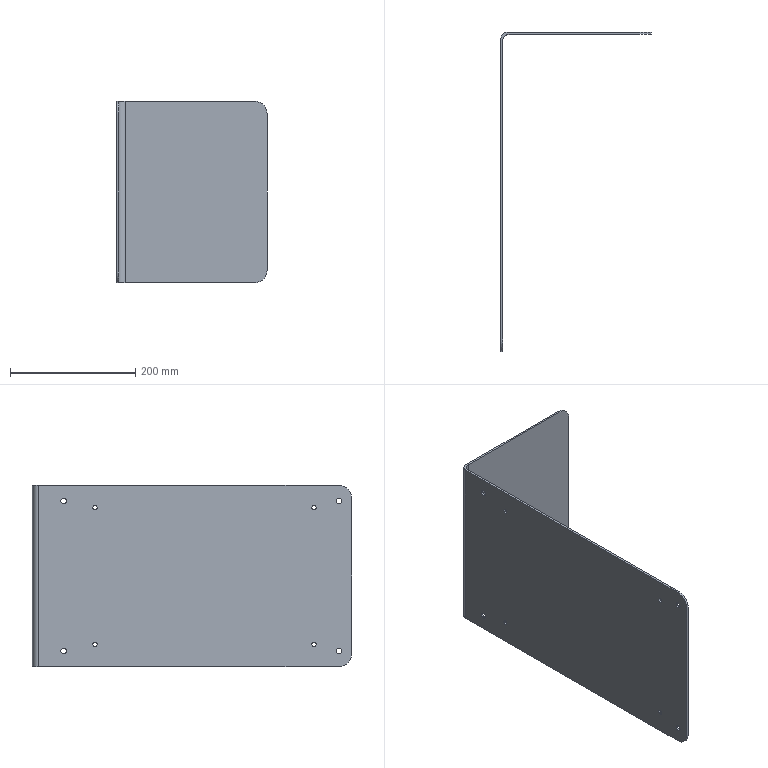Component | SolidWorks | 200-250InverterBracket()-1 | 1 solid | 30 faces | box 240 x 510 x 290 mm | volume 647635 mm3 | cylinder 22 | plane 8 | commonest cylinder face diameters 7 x8 9 x8 40 x4 20 x2 | material Plain Carbon Steel
STEP:
#1=COLOUR_RGB('',0.7922,0.8196,0.9333);
#2=FILL_AREA_STYLE_COLOUR('',#1);
#3=FILL_AREA_STYLE('',(#2));
#4=SURFACE_STYLE_FILL_AREA(#3);
#5=SURFACE_SIDE_STYLE('',(#4));
#6=SURFACE_STYLE_USAGE(.BOTH.,#5);
#7=PRESENTATION_STYLE_ASSIGNMENT((#6));
#8=CARTESIAN_POINT('',(26.575,78.996,-60.669));
#9=VERTEX_POINT('',#8);
#10=CARTESIAN_POINT('',(26.575,79.272,-60.669));
#11=VERTEX_POINT('',#10);
#12=CARTESIAN_POINT('',(26.575,79.134,-60.669));
#13=DIRECTION('',(-1.,0.,-0.));
#14=DIRECTION('',(0.,-1.,0.));
#15=AXIS2_PLACEMENT_3D('',#12,#13,#14);
#16=CIRCLE('',#15,0.1378);
#17=EDGE_CURVE('',#9,#11,#16,.T.);
#18=ORIENTED_EDGE('',*,*,#17,.T.);
#19=CARTESIAN_POINT('',(26.693,79.272,-60.669));
#20=VERTEX_POINT('',#19);
#21=CARTESIAN_POINT('',(26.693,79.272,-60.669));
#22=DIRECTION('',(1.,-0.,0.));
#23=VECTOR('',#22,39.37);
#24=LINE('',#21,#23);
#25=EDGE_CURVE('',#11,#20,#24,.T.);
#26=ORIENTED_EDGE('',*,*,#25,.T.);
#27=CARTESIAN_POINT('',(26.693,78.996,-60.669));
#28=VERTEX_POINT('',#27);
#29=CARTESIAN_POINT('',(26.693,79.134,-60.669));
#30=DIRECTION('',(-1.,0.,-0.));
#31=DIRECTION('',(0.,-1.,0.));
#32=AXIS2_PLACEMENT_3D('',#29,#30,#31);
#33=CIRCLE('',#32,0.1378);
#34=EDGE_CURVE('',#28,#20,#33,.T.);
#35=ORIENTED_EDGE('',*,*,#34,.F.);
#36=CARTESIAN_POINT('',(26.693,78.996,-60.669));
#37=DIRECTION('',(1.,-0.,0.));
#38=VECTOR('',#37,39.37);
#39=LINE('',#36,#38);
#40=EDGE_CURVE('',#9,#28,#39,.T.);
#41=ORIENTED_EDGE('',*,*,#40,.F.);
#42=EDGE_LOOP('',(#18,#26,#35,#41));
#43=FACE_OUTER_BOUND('',#42,.T.);
#44=CARTESIAN_POINT('',(26.693,79.134,-60.669));
#45=DIRECTION('',(1.,-0.,0.));
#46=DIRECTION('',(0.,-1.,0.));
#47=AXIS2_PLACEMENT_3D('',#44,#45,#46);
#48=CYLINDRICAL_SURFACE('',#47,0.1378);
#49=ADVANCED_FACE('',(#43),#48,.F.);
#50=CARTESIAN_POINT('',(26.575,78.996,-69.252));
#51=VERTEX_POINT('',#50);
#52=CARTESIAN_POINT('',(26.575,79.272,-69.252));
#53=VERTEX_POINT('',#52);
#54=CARTESIAN_POINT('',(26.575,79.134,-69.252));
#55=DIRECTION('',(-1.,0.,-0.));
#56=DIRECTION('',(0.,-1.,0.));
#57=AXIS2_PLACEMENT_3D('',#54,#55,#56);
#58=CIRCLE('',#57,0.1378);
#59=EDGE_CURVE('',#51,#53,#58,.T.);
#60=ORIENTED_EDGE('',*,*,#59,.T.);
#61=CARTESIAN_POINT('',(26.693,79.272,-69.252));
#62=VERTEX_POINT('',#61);
#63=CARTESIAN_POINT('',(26.693,79.272,-69.252));
#64=DIRECTION('',(1.,-0.,0.));
#65=VECTOR('',#64,39.37);
#66=LINE('',#63,#65);
#67=EDGE_CURVE('',#53,#62,#66,.T.);
#68=ORIENTED_EDGE('',*,*,#67,.T.);
#69=CARTESIAN_POINT('',(26.693,78.996,-69.252));
#70=VERTEX_POINT('',#69);
#71=CARTESIAN_POINT('',(26.693,79.134,-69.252));
#72=DIRECTION('',(-1.,0.,-0.));
#73=DIRECTION('',(0.,-1.,0.));
#74=AXIS2_PLACEMENT_3D('',#71,#72,#73);
#75=CIRCLE('',#74,0.1378);
#76=EDGE_CURVE('',#70,#62,#75,.T.);
#77=ORIENTED_EDGE('',*,*,#76,.F.);
#78=CARTESIAN_POINT('',(26.693,78.996,-69.252));
#79=DIRECTION('',(1.,-0.,0.));
#80=VECTOR('',#79,39.37);
#81=LINE('',#78,#80);
#82=EDGE_CURVE('',#51,#70,#81,.T.);
#83=ORIENTED_EDGE('',*,*,#82,.F.);
#84=EDGE_LOOP('',(#60,#68,#77,#83));
#85=FACE_OUTER_BOUND('',#84,.T.);
#86=CARTESIAN_POINT('',(26.693,79.134,-69.252));
#87=DIRECTION('',(1.,-0.,0.));
#88=DIRECTION('',(0.,-1.,0.));
#89=AXIS2_PLACEMENT_3D('',#86,#87,#88);
#90=CYLINDRICAL_SURFACE('',#89,0.1378);
#91=ADVANCED_FACE('',(#85),#90,.F.);
#92=CARTESIAN_POINT('',(26.575,92.776,-69.252));
#93=VERTEX_POINT('',#92);
#94=CARTESIAN_POINT('',(26.575,93.051,-69.252));
#95=VERTEX_POINT('',#94);
#96=CARTESIAN_POINT('',(26.575,92.913,-69.252));
#97=DIRECTION('',(-1.,0.,-0.));
#98=DIRECTION('',(0.,-1.,0.));
#99=AXIS2_PLACEMENT_3D('',#96,#97,#98);
#100=CIRCLE('',#99,0.1378);
#101=EDGE_CURVE('',#93,#95,#100,.T.);
#102=ORIENTED_EDGE('',*,*,#101,.T.);
#103=CARTESIAN_POINT('',(26.693,93.051,-69.252));
#104=VERTEX_POINT('',#103);
#105=CARTESIAN_POINT('',(26.693,93.051,-69.252));
#106=DIRECTION('',(1.,-0.,0.));
#107=VECTOR('',#106,39.37);
#108=LINE('',#105,#107);
#109=EDGE_CURVE('',#95,#104,#108,.T.);
#110=ORIENTED_EDGE('',*,*,#109,.T.);
#111=CARTESIAN_POINT('',(26.693,92.776,-69.252));
#112=VERTEX_POINT('',#111);
#113=CARTESIAN_POINT('',(26.693,92.913,-69.252));
#114=DIRECTION('',(-1.,0.,-0.));
#115=DIRECTION('',(0.,-1.,0.));
#116=AXIS2_PLACEMENT_3D('',#113,#114,#115);
#117=CIRCLE('',#116,0.1378);
#118=EDGE_CURVE('',#112,#104,#117,.T.);
#119=ORIENTED_EDGE('',*,*,#118,.F.);
#120=CARTESIAN_POINT('',(26.693,92.776,-69.252));
#121=DIRECTION('',(1.,-0.,0.));
#122=VECTOR('',#121,39.37);
#123=LINE('',#120,#122);
#124=EDGE_CURVE('',#93,#112,#123,.T.);
#125=ORIENTED_EDGE('',*,*,#124,.F.);
#126=EDGE_LOOP('',(#102,#110,#119,#125));
#127=FACE_OUTER_BOUND('',#126,.T.);
#128=CARTESIAN_POINT('',(26.693,92.913,-69.252));
#129=DIRECTION('',(1.,-0.,0.));
#130=DIRECTION('',(0.,-1.,0.));
#131=AXIS2_PLACEMENT_3D('',#128,#129,#130);
#132=CYLINDRICAL_SURFACE('',#131,0.1378);
#133=ADVANCED_FACE('',(#127),#132,.F.);
#134=CARTESIAN_POINT('',(26.575,92.776,-60.669));
#135=VERTEX_POINT('',#134);
#136=CARTESIAN_POINT('',(26.575,93.051,-60.669));
#137=VERTEX_POINT('',#136);
#138=CARTESIAN_POINT('',(26.575,92.913,-60.669));
#139=DIRECTION('',(-1.,0.,-0.));
#140=DIRECTION('',(0.,-1.,0.));
#141=AXIS2_PLACEMENT_3D('',#138,#139,#140);
#142=CIRCLE('',#141,0.1378);
#143=EDGE_CURVE('',#135,#137,#142,.T.);
#144=ORIENTED_EDGE('',*,*,#143,.T.);
#145=CARTESIAN_POINT('',(26.693,93.051,-60.669));
#146=VERTEX_POINT('',#145);
#147=CARTESIAN_POINT('',(26.693,93.051,-60.669));
#148=DIRECTION('',(1.,-0.,0.));
#149=VECTOR('',#148,39.37);
#150=LINE('',#147,#149);
#151=EDGE_CURVE('',#137,#146,#150,.T.);
#152=ORIENTED_EDGE('',*,*,#151,.T.);
#153=CARTESIAN_POINT('',(26.693,92.776,-60.669));
#154=VERTEX_POINT('',#153);
#155=CARTESIAN_POINT('',(26.693,92.913,-60.669));
#156=DIRECTION('',(-1.,0.,-0.));
#157=DIRECTION('',(0.,-1.,0.));
#158=AXIS2_PLACEMENT_3D('',#155,#156,#157);
#159=CIRCLE('',#158,0.1378);
#160=EDGE_CURVE('',#154,#146,#159,.T.);
#161=ORIENTED_EDGE('',*,*,#160,.F.);
#162=CARTESIAN_POINT('',(26.693,92.776,-60.669));
#163=DIRECTION('',(1.,-0.,0.));
#164=VECTOR('',#163,39.37);
#165=LINE('',#162,#164);
#166=EDGE_CURVE('',#135,#154,#165,.T.);
#167=ORIENTED_EDGE('',*,*,#166,.F.);
#168=EDGE_LOOP('',(#144,#152,#161,#167));
#169=FACE_OUTER_BOUND('',#168,.T.);
#170=CARTESIAN_POINT('',(26.693,92.913,-60.669));
#171=DIRECTION('',(1.,-0.,0.));
#172=DIRECTION('',(0.,-1.,0.));
#173=AXIS2_PLACEMENT_3D('',#170,#171,#172);
#174=CYLINDRICAL_SURFACE('',#173,0.1378);
#175=ADVANCED_FACE('',(#169),#174,.F.);
#176=CARTESIAN_POINT('',(26.575,77.382,-69.685));
#177=VERTEX_POINT('',#176);
#178=CARTESIAN_POINT('',(26.575,77.736,-69.685));
#179=VERTEX_POINT('',#178);
#180=CARTESIAN_POINT('',(26.575,77.559,-69.685));
#181=DIRECTION('',(-1.,0.,-0.));
#182=DIRECTION('',(0.,-1.,0.));
#183=AXIS2_PLACEMENT_3D('',#180,#181,#182);
#184=CIRCLE('',#183,0.1772);
#185=EDGE_CURVE('',#177,#179,#184,.T.);
#186=ORIENTED_EDGE('',*,*,#185,.T.);
#187=CARTESIAN_POINT('',(26.693,77.736,-69.685));
#188=VERTEX_POINT('',#187);
#189=CARTESIAN_POINT('',(26.693,77.736,-69.685));
#190=DIRECTION('',(1.,-0.,0.));
#191=VECTOR('',#190,39.37);
#192=LINE('',#189,#191);
#193=EDGE_CURVE('',#179,#188,#192,.T.);
#194=ORIENTED_EDGE('',*,*,#193,.T.);
#195=CARTESIAN_POINT('',(26.693,77.382,-69.685));
#196=VERTEX_POINT('',#195);
#197=CARTESIAN_POINT('',(26.693,77.559,-69.685));
#198=DIRECTION('',(-1.,0.,-0.));
#199=DIRECTION('',(0.,-1.,0.));
#200=AXIS2_PLACEMENT_3D('',#197,#198,#199);
#201=CIRCLE('',#200,0.1772);
#202=EDGE_CURVE('',#196,#188,#201,.T.);
#203=ORIENTED_EDGE('',*,*,#202,.F.);
#204=CARTESIAN_POINT('',(26.693,77.382,-69.685));
#205=DIRECTION('',(1.,-0.,0.));
#206=VECTOR('',#205,39.37);
#207=LINE('',#204,#206);
#208=EDGE_CURVE('',#177,#196,#207,.T.);
#209=ORIENTED_EDGE('',*,*,#208,.F.);
#210=EDGE_LOOP('',(#186,#194,#203,#209));
#211=FACE_OUTER_BOUND('',#210,.T.);
#212=CARTESIAN_POINT('',(26.693,77.559,-69.685));
#213=DIRECTION('',(1.,-0.,0.));
#214=DIRECTION('',(0.,-1.,0.));
#215=AXIS2_PLACEMENT_3D('',#212,#213,#214);
#216=CYLINDRICAL_SURFACE('',#215,0.1772);
#217=ADVANCED_FACE('',(#211),#216,.F.);
#218=CARTESIAN_POINT('',(26.575,77.382,-60.236));
#219=VERTEX_POINT('',#218);
#220=CARTESIAN_POINT('',(26.575,77.736,-60.236));
#221=VERTEX_POINT('',#220);
#222=CARTESIAN_POINT('',(26.575,77.559,-60.236));
#223=DIRECTION('',(-1.,0.,-0.));
#224=DIRECTION('',(0.,-1.,0.));
#225=AXIS2_PLACEMENT_3D('',#222,#223,#224);
#226=CIRCLE('',#225,0.1772);
#227=EDGE_CURVE('',#219,#221,#226,.T.);
#228=ORIENTED_EDGE('',*,*,#227,.T.);
#229=CARTESIAN_POINT('',(26.693,77.736,-60.236));
#230=VERTEX_POINT('',#229);
#231=CARTESIAN_POINT('',(26.693,77.736,-60.236));
#232=DIRECTION('',(1.,-0.,0.));
#233=VECTOR('',#232,39.37);
#234=LINE('',#231,#233);
#235=EDGE_CURVE('',#221,#230,#234,.T.);
#236=ORIENTED_EDGE('',*,*,#235,.T.);
#237=CARTESIAN_POINT('',(26.693,77.382,-60.236));
#238=VERTEX_POINT('',#237);
#239=CARTESIAN_POINT('',(26.693,77.559,-60.236));
#240=DIRECTION('',(-1.,0.,-0.));
#241=DIRECTION('',(0.,-1.,0.));
#242=AXIS2_PLACEMENT_3D('',#239,#240,#241);
#243=CIRCLE('',#242,0.1772);
#244=EDGE_CURVE('',#238,#230,#243,.T.);
#245=ORIENTED_EDGE('',*,*,#244,.F.);
#246=CARTESIAN_POINT('',(26.693,77.382,-60.236));
#247=DIRECTION('',(1.,-0.,0.));
#248=VECTOR('',#247,39.37);
#249=LINE('',#246,#248);
#250=EDGE_CURVE('',#219,#238,#249,.T.);
#251=ORIENTED_EDGE('',*,*,#250,.F.);
#252=EDGE_LOOP('',(#228,#236,#245,#251));
#253=FACE_OUTER_BOUND('',#252,.T.);
#254=CARTESIAN_POINT('',(26.693,77.559,-60.236));
#255=DIRECTION('',(1.,-0.,0.));
#256=DIRECTION('',(0.,-1.,0.));
#257=AXIS2_PLACEMENT_3D('',#254,#255,#256);
#258=CYLINDRICAL_SURFACE('',#257,0.1772);
#259=ADVANCED_FACE('',(#253),#258,.F.);
#260=CARTESIAN_POINT('',(26.575,94.705,-60.236));
#261=VERTEX_POINT('',#260);
#262=CARTESIAN_POINT('',(26.575,95.059,-60.236));
#263=VERTEX_POINT('',#262);
#264=CARTESIAN_POINT('',(26.575,94.882,-60.236));
#265=DIRECTION('',(-1.,0.,-0.));
#266=DIRECTION('',(0.,-1.,0.));
#267=AXIS2_PLACEMENT_3D('',#264,#265,#266);
#268=CIRCLE('',#267,0.1772);
#269=EDGE_CURVE('',#261,#263,#268,.T.);
#270=ORIENTED_EDGE('',*,*,#269,.T.);
#271=CARTESIAN_POINT('',(26.693,95.059,-60.236));
#272=VERTEX_POINT('',#271);
#273=CARTESIAN_POINT('',(26.693,95.059,-60.236));
#274=DIRECTION('',(1.,-0.,0.));
#275=VECTOR('',#274,39.37);
#276=LINE('',#273,#275);
#277=EDGE_CURVE('',#263,#272,#276,.T.);
#278=ORIENTED_EDGE('',*,*,#277,.T.);
#279=CARTESIAN_POINT('',(26.693,94.705,-60.236));
#280=VERTEX_POINT('',#279);
#281=CARTESIAN_POINT('',(26.693,94.882,-60.236));
#282=DIRECTION('',(-1.,0.,-0.));
#283=DIRECTION('',(0.,-1.,0.));
#284=AXIS2_PLACEMENT_3D('',#281,#282,#283);
#285=CIRCLE('',#284,0.1772);
#286=EDGE_CURVE('',#280,#272,#285,.T.);
#287=ORIENTED_EDGE('',*,*,#286,.F.);
#288=CARTESIAN_POINT('',(26.693,94.705,-60.236));
#289=DIRECTION('',(1.,-0.,0.));
#290=VECTOR('',#289,39.37);
#291=LINE('',#288,#290);
#292=EDGE_CURVE('',#261,#280,#291,.T.);
#293=ORIENTED_EDGE('',*,*,#292,.F.);
#294=EDGE_LOOP('',(#270,#278,#287,#293));
#295=FACE_OUTER_BOUND('',#294,.T.);
#296=CARTESIAN_POINT('',(26.693,94.882,-60.236));
#297=DIRECTION('',(1.,-0.,0.));
#298=DIRECTION('',(0.,-1.,0.));
#299=AXIS2_PLACEMENT_3D('',#296,#297,#298);
#300=CYLINDRICAL_SURFACE('',#299,0.1772);
#301=ADVANCED_FACE('',(#295),#300,.F.);
#302=CARTESIAN_POINT('',(26.575,94.705,-69.685));
#303=VERTEX_POINT('',#302);
#304=CARTESIAN_POINT('',(26.575,95.059,-69.685));
#305=VERTEX_POINT('',#304);
#306=CARTESIAN_POINT('',(26.575,94.882,-69.685));
#307=DIRECTION('',(-1.,0.,-0.));
#308=DIRECTION('',(0.,-1.,0.));
#309=AXIS2_PLACEMENT_3D('',#306,#307,#308);
#310=CIRCLE('',#309,0.1772);
#311=EDGE_CURVE('',#303,#305,#310,.T.);
#312=ORIENTED_EDGE('',*,*,#311,.T.);
#313=CARTESIAN_POINT('',(26.693,95.059,-69.685));
#314=VERTEX_POINT('',#313);
#315=CARTESIAN_POINT('',(26.693,95.059,-69.685));
#316=DIRECTION('',(1.,-0.,0.));
#317=VECTOR('',#316,39.37);
#318=LINE('',#315,#317);
#319=EDGE_CURVE('',#305,#314,#318,.T.);
#320=ORIENTED_EDGE('',*,*,#319,.T.);
#321=CARTESIAN_POINT('',(26.693,94.705,-69.685));
#322=VERTEX_POINT('',#321);
#323=CARTESIAN_POINT('',(26.693,94.882,-69.685));
#324=DIRECTION('',(-1.,0.,-0.));
#325=DIRECTION('',(0.,-1.,0.));
#326=AXIS2_PLACEMENT_3D('',#323,#324,#325);
#327=CIRCLE('',#326,0.1772);
#328=EDGE_CURVE('',#322,#314,#327,.T.);
#329=ORIENTED_EDGE('',*,*,#328,.F.);
#330=CARTESIAN_POINT('',(26.693,94.705,-69.685));
#331=DIRECTION('',(1.,-0.,0.));
#332=VECTOR('',#331,39.37);
#333=LINE('',#330,#332);
#334=EDGE_CURVE('',#303,#322,#333,.T.);
#335=ORIENTED_EDGE('',*,*,#334,.F.);
#336=EDGE_LOOP('',(#312,#320,#329,#335));
#337=FACE_OUTER_BOUND('',#336,.T.);
#338=CARTESIAN_POINT('',(26.693,94.882,-69.685));
#339=DIRECTION('',(1.,-0.,0.));
#340=DIRECTION('',(0.,-1.,0.));
#341=AXIS2_PLACEMENT_3D('',#338,#339,#340);
#342=CYLINDRICAL_SURFACE('',#341,0.1772);
#343=ADVANCED_FACE('',(#337),#342,.F.);
#344=CARTESIAN_POINT('',(26.575,76.772,-69.882));
#345=VERTEX_POINT('',#344);
#346=CARTESIAN_POINT('',(26.575,77.559,-70.669));
#347=VERTEX_POINT('',#346);
#348=CARTESIAN_POINT('',(26.575,77.559,-69.882));
#349=DIRECTION('',(1.,-0.,0.));
#350=DIRECTION('',(0.,-1.,0.));
#351=AXIS2_PLACEMENT_3D('',#348,#349,#350);
#352=CIRCLE('',#351,0.7874);
#353=EDGE_CURVE('',#345,#347,#352,.T.);
#354=ORIENTED_EDGE('',*,*,#353,.F.);
#355=CARTESIAN_POINT('',(26.575,76.772,-60.039));
#356=VERTEX_POINT('',#355);
#357=CARTESIAN_POINT('',(26.575,76.772,-70.669));
#358=DIRECTION('',(0.,0.,-1.));
#359=VECTOR('',#358,39.37);
#360=LINE('',#357,#359);
#361=EDGE_CURVE('',#356,#345,#360,.T.);
#362=ORIENTED_EDGE('',*,*,#361,.F.);
#363=CARTESIAN_POINT('',(26.575,77.559,-59.252));
#364=VERTEX_POINT('',#363);
#365=CARTESIAN_POINT('',(26.575,77.559,-60.039));
#366=DIRECTION('',(1.,-0.,0.));
#367=DIRECTION('',(0.,1.,0.));
#368=AXIS2_PLACEMENT_3D('',#365,#366,#367);
#369=CIRCLE('',#368,0.7874);
#370=EDGE_CURVE('',#364,#356,#369,.T.);
#371=ORIENTED_EDGE('',*,*,#370,.F.);
#372=CARTESIAN_POINT('',(26.575,96.457,-59.252));
#373=VERTEX_POINT('',#372);
#374=CARTESIAN_POINT('',(26.575,76.772,-59.252));
#375=DIRECTION('',(-0.,-1.,-0.));
#376=VECTOR('',#375,39.37);
#377=LINE('',#374,#376);
#378=EDGE_CURVE('',#373,#364,#377,.T.);
#379=ORIENTED_EDGE('',*,*,#378,.F.);
#380=CARTESIAN_POINT('',(26.575,96.457,-70.669));
#381=VERTEX_POINT('',#380);
#382=CARTESIAN_POINT('',(26.575,96.457,-70.669));
#383=DIRECTION('',(-0.,-0.,1.));
#384=VECTOR('',#383,39.37);
#385=LINE('',#382,#384);
#386=EDGE_CURVE('',#381,#373,#385,.T.);
#387=ORIENTED_EDGE('',*,*,#386,.F.);
#388=CARTESIAN_POINT('',(26.575,76.772,-70.669));
#389=DIRECTION('',(0.,1.,0.));
#390=VECTOR('',#389,39.37);
#391=LINE('',#388,#390);
#392=EDGE_CURVE('',#347,#381,#391,.T.);
#393=ORIENTED_EDGE('',*,*,#392,.F.);
#394=EDGE_LOOP('',(#354,#362,#371,#379,#387,#393));
#395=FACE_OUTER_BOUND('',#394,.T.);
#396=ORIENTED_EDGE('',*,*,#17,.F.);
#397=CARTESIAN_POINT('',(26.575,79.134,-60.669));
#398=DIRECTION('',(-1.,0.,-0.));
#399=DIRECTION('',(0.,-1.,0.));
#400=AXIS2_PLACEMENT_3D('',#397,#398,#399);
#401=CIRCLE('',#400,0.1378);
#402=EDGE_CURVE('',#11,#9,#401,.T.);
#403=ORIENTED_EDGE('',*,*,#402,.F.);
#404=EDGE_LOOP('',(#396,#403));
#405=FACE_BOUND('',#404,.T.);
#406=ORIENTED_EDGE('',*,*,#59,.F.);
#407=CARTESIAN_POINT('',(26.575,79.134,-69.252));
#408=DIRECTION('',(-1.,0.,-0.));
#409=DIRECTION('',(0.,-1.,0.));
#410=AXIS2_PLACEMENT_3D('',#407,#408,#409);
#411=CIRCLE('',#410,0.1378);
#412=EDGE_CURVE('',#53,#51,#411,.T.);
#413=ORIENTED_EDGE('',*,*,#412,.F.);
#414=EDGE_LOOP('',(#406,#413));
#415=FACE_BOUND('',#414,.T.);
#416=ORIENTED_EDGE('',*,*,#101,.F.);
#417=CARTESIAN_POINT('',(26.575,92.913,-69.252));
#418=DIRECTION('',(-1.,0.,-0.));
#419=DIRECTION('',(0.,-1.,0.));
#420=AXIS2_PLACEMENT_3D('',#417,#418,#419);
#421=CIRCLE('',#420,0.1378);
#422=EDGE_CURVE('',#95,#93,#421,.T.);
#423=ORIENTED_EDGE('',*,*,#422,.F.);
#424=EDGE_LOOP('',(#416,#423));
#425=FACE_BOUND('',#424,.T.);
#426=ORIENTED_EDGE('',*,*,#143,.F.);
#427=CARTESIAN_POINT('',(26.575,92.913,-60.669));
#428=DIRECTION('',(-1.,0.,-0.));
#429=DIRECTION('',(0.,-1.,0.));
#430=AXIS2_PLACEMENT_3D('',#427,#428,#429);
#431=CIRCLE('',#430,0.1378);
#432=EDGE_CURVE('',#137,#135,#431,.T.);
#433=ORIENTED_EDGE('',*,*,#432,.F.);
#434=EDGE_LOOP('',(#426,#433));
#435=FACE_BOUND('',#434,.T.);
#436=ORIENTED_EDGE('',*,*,#185,.F.);
#437=CARTESIAN_POINT('',(26.575,77.559,-69.685));
#438=DIRECTION('',(-1.,0.,-0.));
#439=DIRECTION('',(0.,-1.,0.));
#440=AXIS2_PLACEMENT_3D('',#437,#438,#439);
#441=CIRCLE('',#440,0.1772);
#442=EDGE_CURVE('',#179,#177,#441,.T.);
#443=ORIENTED_EDGE('',*,*,#442,.F.);
#444=EDGE_LOOP('',(#436,#443));
#445=FACE_BOUND('',#444,.T.);
#446=ORIENTED_EDGE('',*,*,#227,.F.);
#447=CARTESIAN_POINT('',(26.575,77.559,-60.236));
#448=DIRECTION('',(-1.,0.,-0.));
#449=DIRECTION('',(0.,-1.,0.));
#450=AXIS2_PLACEMENT_3D('',#447,#448,#449);
#451=CIRCLE('',#450,0.1772);
#452=EDGE_CURVE('',#221,#219,#451,.T.);
#453=ORIENTED_EDGE('',*,*,#452,.F.);
#454=EDGE_LOOP('',(#446,#453));
#455=FACE_BOUND('',#454,.T.);
#456=ORIENTED_EDGE('',*,*,#269,.F.);
#457=CARTESIAN_POINT('',(26.575,94.882,-60.236));
#458=DIRECTION('',(-1.,0.,-0.));
#459=DIRECTION('',(0.,-1.,0.));
#460=AXIS2_PLACEMENT_3D('',#457,#458,#459);
#461=CIRCLE('',#460,0.1772);
#462=EDGE_CURVE('',#263,#261,#461,.T.);
#463=ORIENTED_EDGE('',*,*,#462,.F.);
#464=EDGE_LOOP('',(#456,#463));
#465=FACE_BOUND('',#464,.T.);
#466=ORIENTED_EDGE('',*,*,#311,.F.);
#467=CARTESIAN_POINT('',(26.575,94.882,-69.685));
#468=DIRECTION('',(-1.,0.,-0.));
#469=DIRECTION('',(0.,-1.,0.));
#470=AXIS2_PLACEMENT_3D('',#467,#468,#469);
#471=CIRCLE('',#470,0.1772);
#472=EDGE_CURVE('',#305,#303,#471,.T.);
#473=ORIENTED_EDGE('',*,*,#472,.F.);
#474=EDGE_LOOP('',(#466,#473));
#475=FACE_BOUND('',#474,.T.);
#476=CARTESIAN_POINT('',(26.575,76.772,-70.669));
#477=DIRECTION('',(1.,-0.,0.));
#478=DIRECTION('',(-0.,-1.,-0.));
#479=AXIS2_PLACEMENT_3D('',#476,#477,#478);
#480=PLANE('',#479);
#481=ADVANCED_FACE('',(#395,#405,#415,#425,#435,#445,#455,#465,#475),#480,.F.);
#482=CARTESIAN_POINT('',(35.236,96.732,-70.669));
#483=VERTEX_POINT('',#482);
#484=CARTESIAN_POINT('',(27.087,96.732,-70.669));
#485=VERTEX_POINT('',#484);
#486=CARTESIAN_POINT('',(26.969,96.732,-70.669));
#487=DIRECTION('',(-1.,0.,-0.));
#488=VECTOR('',#487,39.37);
#489=LINE('',#486,#488);
#490=EDGE_CURVE('',#483,#485,#489,.T.);
#491=ORIENTED_EDGE('',*,*,#490,.T.);
#492=CARTESIAN_POINT('',(26.693,96.339,-70.669));
#493=VERTEX_POINT('',#492);
#494=CARTESIAN_POINT('',(27.087,96.339,-70.669));
#495=DIRECTION('',(-0.,-0.,1.));
#496=DIRECTION('',(0.,1.,0.));
#497=AXIS2_PLACEMENT_3D('',#494,#495,#496);
#498=CIRCLE('',#497,0.3937);
#499=EDGE_CURVE('',#485,#493,#498,.T.);
#500=ORIENTED_EDGE('',*,*,#499,.T.);
#501=CARTESIAN_POINT('',(26.693,77.559,-70.669));
#502=VERTEX_POINT('',#501);
#503=CARTESIAN_POINT('',(26.693,96.457,-70.669));
#504=DIRECTION('',(-0.,-1.,-0.));
#505=VECTOR('',#504,39.37);
#506=LINE('',#503,#505);
#507=EDGE_CURVE('',#493,#502,#506,.T.);
#508=ORIENTED_EDGE('',*,*,#507,.T.);
#509=CARTESIAN_POINT('',(26.969,77.559,-70.669));
#510=DIRECTION('',(-1.,0.,-0.));
#511=VECTOR('',#510,39.37);
#512=LINE('',#509,#511);
#513=EDGE_CURVE('',#502,#347,#512,.T.);
#514=ORIENTED_EDGE('',*,*,#513,.T.);
#515=ORIENTED_EDGE('',*,*,#392,.T.);
#516=CARTESIAN_POINT('',(26.969,96.85,-70.669));
#517=VERTEX_POINT('',#516);
#518=CARTESIAN_POINT('',(26.969,96.457,-70.669));
#519=DIRECTION('',(0.,0.,-1.));
#520=DIRECTION('',(0.,1.,0.));
#521=AXIS2_PLACEMENT_3D('',#518,#519,#520);
#522=CIRCLE('',#521,0.3937);
#523=EDGE_CURVE('',#381,#517,#522,.T.);
#524=ORIENTED_EDGE('',*,*,#523,.T.);
#525=CARTESIAN_POINT('',(35.236,96.85,-70.669));
#526=VERTEX_POINT('',#525);
#527=CARTESIAN_POINT('',(26.969,96.85,-70.669));
#528=DIRECTION('',(1.,-0.,0.));
#529=VECTOR('',#528,39.37);
#530=LINE('',#527,#529);
#531=EDGE_CURVE('',#517,#526,#530,.T.);
#532=ORIENTED_EDGE('',*,*,#531,.T.);
#533=CARTESIAN_POINT('',(35.236,96.457,-70.669));
#534=DIRECTION('',(-0.,-1.,-0.));
#535=VECTOR('',#534,39.37);
#536=LINE('',#533,#535);
#537=EDGE_CURVE('',#526,#483,#536,.T.);
#538=ORIENTED_EDGE('',*,*,#537,.T.);
#539=EDGE_LOOP('',(#491,#500,#508,#514,#515,#524,#532,#538));
#540=FACE_OUTER_BOUND('',#539,.T.);
#541=CARTESIAN_POINT('',(26.969,96.457,-70.669));
#542=DIRECTION('',(0.,0.,-1.));
#543=DIRECTION('',(-0.,-1.,-0.));
#544=AXIS2_PLACEMENT_3D('',#541,#542,#543);
#545=PLANE('',#544);
#546=ADVANCED_FACE('',(#540),#545,.T.);
#547=ORIENTED_EDGE('',*,*,#353,.T.);
#548=ORIENTED_EDGE('',*,*,#513,.F.);
#549=CARTESIAN_POINT('',(26.693,76.772,-69.882));
#550=VERTEX_POINT('',#549);
#551=CARTESIAN_POINT('',(26.693,77.559,-69.882));
#552=DIRECTION('',(-1.,0.,-0.));
#553=DIRECTION('',(0.,-1.,0.));
#554=AXIS2_PLACEMENT_3D('',#551,#552,#553);
#555=CIRCLE('',#554,0.7874);
#556=EDGE_CURVE('',#502,#550,#555,.T.);
#557=ORIENTED_EDGE('',*,*,#556,.T.);
#558=CARTESIAN_POINT('',(26.969,76.772,-69.882));
#559=DIRECTION('',(-1.,0.,-0.));
#560=VECTOR('',#559,39.37);
#561=LINE('',#558,#560);
#562=EDGE_CURVE('',#550,#345,#561,.T.);
#563=ORIENTED_EDGE('',*,*,#562,.T.);
#564=EDGE_LOOP('',(#547,#548,#557,#563));
#565=FACE_OUTER_BOUND('',#564,.T.);
#566=CARTESIAN_POINT('',(26.969,77.559,-69.882));
#567=DIRECTION('',(1.,-0.,0.));
#568=DIRECTION('',(0.,-1.,0.));
#569=AXIS2_PLACEMENT_3D('',#566,#567,#568);
#570=CYLINDRICAL_SURFACE('',#569,0.7874);
#571=ADVANCED_FACE('',(#565),#570,.T.);
#572=ORIENTED_EDGE('',*,*,#562,.F.);
#573=CARTESIAN_POINT('',(26.693,76.772,-60.039));
#574=VERTEX_POINT('',#573);
#575=CARTESIAN_POINT('',(26.693,76.772,-70.669));
#576=DIRECTION('',(0.,0.,-1.));
#577=VECTOR('',#576,39.37);
#578=LINE('',#575,#577);
#579=EDGE_CURVE('',#574,#550,#578,.T.);
#580=ORIENTED_EDGE('',*,*,#579,.F.);
#581=CARTESIAN_POINT('',(26.693,76.772,-60.039));
#582=DIRECTION('',(1.,-0.,0.));
#583=VECTOR('',#582,39.37);
#584=LINE('',#581,#583);
#585=EDGE_CURVE('',#356,#574,#584,.T.);
#586=ORIENTED_EDGE('',*,*,#585,.F.);
#587=ORIENTED_EDGE('',*,*,#361,.T.);
#588=EDGE_LOOP('',(#572,#580,#586,#587));
#589=FACE_OUTER_BOUND('',#588,.T.);
#590=CARTESIAN_POINT('',(26.693,76.772,-70.669));
#591=DIRECTION('',(0.,1.,0.));
#592=DIRECTION('',(1.,-0.,0.));
#593=AXIS2_PLACEMENT_3D('',#590,#591,#592);
#594=PLANE('',#593);
#595=ADVANCED_FACE('',(#589),#594,.F.);
#596=ORIENTED_EDGE('',*,*,#370,.T.);
#597=ORIENTED_EDGE('',*,*,#585,.T.);
#598=CARTESIAN_POINT('',(26.693,77.559,-59.252));
#599=VERTEX_POINT('',#598);
#600=CARTESIAN_POINT('',(26.693,77.559,-60.039));
#601=DIRECTION('',(-1.,0.,-0.));
#602=DIRECTION('',(0.,1.,0.));
#603=AXIS2_PLACEMENT_3D('',#600,#601,#602);
#604=CIRCLE('',#603,0.7874);
#605=EDGE_CURVE('',#574,#599,#604,.T.);
#606=ORIENTED_EDGE('',*,*,#605,.T.);
#607=CARTESIAN_POINT('',(26.693,77.559,-59.252));
#608=DIRECTION('',(-1.,0.,-0.));
#609=VECTOR('',#608,39.37);
#610=LINE('',#607,#609);
#611=EDGE_CURVE('',#599,#364,#610,.T.);
#612=ORIENTED_EDGE('',*,*,#611,.T.);
#613=EDGE_LOOP('',(#596,#597,#606,#612));
#614=FACE_OUTER_BOUND('',#613,.T.);
#615=CARTESIAN_POINT('',(26.693,77.559,-60.039));
#616=DIRECTION('',(-1.,0.,-0.));
#617=DIRECTION('',(0.,1.,0.));
#618=AXIS2_PLACEMENT_3D('',#615,#616,#617);
#619=CYLINDRICAL_SURFACE('',#618,0.7874);
#620=ADVANCED_FACE('',(#614),#619,.T.);
#621=ORIENTED_EDGE('',*,*,#611,.F.);
#622=CARTESIAN_POINT('',(26.693,96.339,-59.252));
#623=VERTEX_POINT('',#622);
#624=CARTESIAN_POINT('',(26.693,96.457,-59.252));
#625=DIRECTION('',(-0.,-1.,-0.));
#626=VECTOR('',#625,39.37);
#627=LINE('',#624,#626);
#628=EDGE_CURVE('',#623,#599,#627,.T.);
#629=ORIENTED_EDGE('',*,*,#628,.F.);
#630=CARTESIAN_POINT('',(27.087,96.732,-59.252));
#631=VERTEX_POINT('',#630);
#632=CARTESIAN_POINT('',(27.087,96.339,-59.252));
#633=DIRECTION('',(-0.,-0.,1.));
#634=DIRECTION('',(0.,1.,0.));
#635=AXIS2_PLACEMENT_3D('',#632,#633,#634);
#636=CIRCLE('',#635,0.3937);
#637=EDGE_CURVE('',#631,#623,#636,.T.);
#638=ORIENTED_EDGE('',*,*,#637,.F.);
#639=CARTESIAN_POINT('',(35.236,96.732,-59.252));
#640=VERTEX_POINT('',#639);
#641=CARTESIAN_POINT('',(26.969,96.732,-59.252));
#642=DIRECTION('',(-1.,0.,-0.));
#643=VECTOR('',#642,39.37);
#644=LINE('',#641,#643);
#645=EDGE_CURVE('',#640,#631,#644,.T.);
#646=ORIENTED_EDGE('',*,*,#645,.F.);
#647=CARTESIAN_POINT('',(35.236,96.85,-59.252));
#648=VERTEX_POINT('',#647);
#649=CARTESIAN_POINT('',(35.236,96.457,-59.252));
#650=DIRECTION('',(-0.,-1.,-0.));
#651=VECTOR('',#650,39.37);
#652=LINE('',#649,#651);
#653=EDGE_CURVE('',#648,#640,#652,.T.);
#654=ORIENTED_EDGE('',*,*,#653,.F.);
#655=CARTESIAN_POINT('',(26.969,96.85,-59.252));
#656=VERTEX_POINT('',#655);
#657=CARTESIAN_POINT('',(26.969,96.85,-59.252));
#658=DIRECTION('',(1.,-0.,0.));
#659=VECTOR('',#658,39.37);
#660=LINE('',#657,#659);
#661=EDGE_CURVE('',#656,#648,#660,.T.);
#662=ORIENTED_EDGE('',*,*,#661,.F.);
#663=CARTESIAN_POINT('',(26.969,96.457,-59.252));
#664=DIRECTION('',(0.,0.,-1.));
#665=DIRECTION('',(0.,1.,0.));
#666=AXIS2_PLACEMENT_3D('',#663,#664,#665);
#667=CIRCLE('',#666,0.3937);
#668=EDGE_CURVE('',#373,#656,#667,.T.);
#669=ORIENTED_EDGE('',*,*,#668,.F.);
#670=ORIENTED_EDGE('',*,*,#378,.T.);
#671=EDGE_LOOP('',(#621,#629,#638,#646,#654,#662,#669,#670));
#672=FACE_OUTER_BOUND('',#671,.T.);
#673=CARTESIAN_POINT('',(26.969,96.457,-59.252));
#674=DIRECTION('',(0.,0.,-1.));
#675=DIRECTION('',(-0.,-1.,-0.));
#676=AXIS2_PLACEMENT_3D('',#673,#674,#675);
#677=PLANE('',#676);
#678=ADVANCED_FACE('',(#672),#677,.F.);
#679=ORIENTED_EDGE('',*,*,#523,.F.);
#680=ORIENTED_EDGE('',*,*,#386,.T.);
#681=ORIENTED_EDGE('',*,*,#668,.T.);
#682=CARTESIAN_POINT('',(26.969,96.85,-70.669));
#683=DIRECTION('',(0.,0.,-1.));
#684=VECTOR('',#683,39.37);
#685=LINE('',#682,#684);
#686=EDGE_CURVE('',#656,#517,#685,.T.);
#687=ORIENTED_EDGE('',*,*,#686,.T.);
#688=EDGE_LOOP('',(#679,#680,#681,#687));
#689=FACE_OUTER_BOUND('',#688,.T.);
#690=CARTESIAN_POINT('',(26.969,96.457,-70.669));
#691=DIRECTION('',(-0.,-0.,1.));
#692=DIRECTION('',(0.,1.,0.));
#693=AXIS2_PLACEMENT_3D('',#690,#691,#692);
#694=CYLINDRICAL_SURFACE('',#693,0.3937);
#695=ADVANCED_FACE('',(#689),#694,.T.);
#696=ORIENTED_EDGE('',*,*,#25,.F.);
#697=ORIENTED_EDGE('',*,*,#402,.T.);
#698=ORIENTED_EDGE('',*,*,#40,.T.);
#699=CARTESIAN_POINT('',(26.693,79.134,-60.669));
#700=DIRECTION('',(-1.,0.,-0.));
#701=DIRECTION('',(0.,-1.,0.));
#702=AXIS2_PLACEMENT_3D('',#699,#700,#701);
#703=CIRCLE('',#702,0.1378);
#704=EDGE_CURVE('',#20,#28,#703,.T.);
#705=ORIENTED_EDGE('',*,*,#704,.F.);
#706=EDGE_LOOP('',(#696,#697,#698,#705));
#707=FACE_OUTER_BOUND('',#706,.T.);
#708=CARTESIAN_POINT('',(26.693,79.134,-60.669));
#709=DIRECTION('',(1.,-0.,0.));
#710=DIRECTION('',(0.,-1.,0.));
#711=AXIS2_PLACEMENT_3D('',#708,#709,#710);
#712=CYLINDRICAL_SURFACE('',#711,0.1378);
#713=ADVANCED_FACE('',(#707),#712,.F.);
#714=ORIENTED_EDGE('',*,*,#67,.F.);
#715=ORIENTED_EDGE('',*,*,#412,.T.);
#716=ORIENTED_EDGE('',*,*,#82,.T.);
#717=CARTESIAN_POINT('',(26.693,79.134,-69.252));
#718=DIRECTION('',(-1.,0.,-0.));
#719=DIRECTION('',(0.,-1.,0.));
#720=AXIS2_PLACEMENT_3D('',#717,#718,#719);
#721=CIRCLE('',#720,0.1378);
#722=EDGE_CURVE('',#62,#70,#721,.T.);
#723=ORIENTED_EDGE('',*,*,#722,.F.);
#724=EDGE_LOOP('',(#714,#715,#716,#723));
#725=FACE_OUTER_BOUND('',#724,.T.);
#726=CARTESIAN_POINT('',(26.693,79.134,-69.252));
#727=DIRECTION('',(1.,-0.,0.));
#728=DIRECTION('',(0.,-1.,0.));
#729=AXIS2_PLACEMENT_3D('',#726,#727,#728);
#730=CYLINDRICAL_SURFACE('',#729,0.1378);
#731=ADVANCED_FACE('',(#725),#730,.F.);
#732=ORIENTED_EDGE('',*,*,#109,.F.);
#733=ORIENTED_EDGE('',*,*,#422,.T.);
#734=ORIENTED_EDGE('',*,*,#124,.T.);
#735=CARTESIAN_POINT('',(26.693,92.913,-69.252));
#736=DIRECTION('',(-1.,0.,-0.));
#737=DIRECTION('',(0.,-1.,0.));
#738=AXIS2_PLACEMENT_3D('',#735,#736,#737);
#739=CIRCLE('',#738,0.1378);
#740=EDGE_CURVE('',#104,#112,#739,.T.);
#741=ORIENTED_EDGE('',*,*,#740,.F.);
#742=EDGE_LOOP('',(#732,#733,#734,#741));
#743=FACE_OUTER_BOUND('',#742,.T.);
#744=CARTESIAN_POINT('',(26.693,92.913,-69.252));
#745=DIRECTION('',(1.,-0.,0.));
#746=DIRECTION('',(0.,-1.,0.));
#747=AXIS2_PLACEMENT_3D('',#744,#745,#746);
#748=CYLINDRICAL_SURFACE('',#747,0.1378);
#749=ADVANCED_FACE('',(#743),#748,.F.);
#750=ORIENTED_EDGE('',*,*,#151,.F.);
#751=ORIENTED_EDGE('',*,*,#432,.T.);
#752=ORIENTED_EDGE('',*,*,#166,.T.);
#753=CARTESIAN_POINT('',(26.693,92.913,-60.669));
#754=DIRECTION('',(-1.,0.,-0.));
#755=DIRECTION('',(0.,-1.,0.));
#756=AXIS2_PLACEMENT_3D('',#753,#754,#755);
#757=CIRCLE('',#756,0.1378);
#758=EDGE_CURVE('',#146,#154,#757,.T.);
#759=ORIENTED_EDGE('',*,*,#758,.F.);
#760=EDGE_LOOP('',(#750,#751,#752,#759));
#761=FACE_OUTER_BOUND('',#760,.T.);
#762=CARTESIAN_POINT('',(26.693,92.913,-60.669));
#763=DIRECTION('',(1.,-0.,0.));
#764=DIRECTION('',(0.,-1.,0.));
#765=AXIS2_PLACEMENT_3D('',#762,#763,#764);
#766=CYLINDRICAL_SURFACE('',#765,0.1378);
#767=ADVANCED_FACE('',(#761),#766,.F.);
#768=ORIENTED_EDGE('',*,*,#193,.F.);
#769=ORIENTED_EDGE('',*,*,#442,.T.);
#770=ORIENTED_EDGE('',*,*,#208,.T.);
#771=CARTESIAN_POINT('',(26.693,77.559,-69.685));
#772=DIRECTION('',(-1.,0.,-0.));
#773=DIRECTION('',(0.,-1.,0.));
#774=AXIS2_PLACEMENT_3D('',#771,#772,#773);
#775=CIRCLE('',#774,0.1772);
#776=EDGE_CURVE('',#188,#196,#775,.T.);
#777=ORIENTED_EDGE('',*,*,#776,.F.);
#778=EDGE_LOOP('',(#768,#769,#770,#777));
#779=FACE_OUTER_BOUND('',#778,.T.);
#780=CARTESIAN_POINT('',(26.693,77.559,-69.685));
#781=DIRECTION('',(1.,-0.,0.));
#782=DIRECTION('',(0.,-1.,0.));
#783=AXIS2_PLACEMENT_3D('',#780,#781,#782);
#784=CYLINDRICAL_SURFACE('',#783,0.1772);
#785=ADVANCED_FACE('',(#779),#784,.F.);
#786=ORIENTED_EDGE('',*,*,#235,.F.);
#787=ORIENTED_EDGE('',*,*,#452,.T.);
#788=ORIENTED_EDGE('',*,*,#250,.T.);
#789=CARTESIAN_POINT('',(26.693,77.559,-60.236));
#790=DIRECTION('',(-1.,0.,-0.));
#791=DIRECTION('',(0.,-1.,0.));
#792=AXIS2_PLACEMENT_3D('',#789,#790,#791);
#793=CIRCLE('',#792,0.1772);
#794=EDGE_CURVE('',#230,#238,#793,.T.);
#795=ORIENTED_EDGE('',*,*,#794,.F.);
#796=EDGE_LOOP('',(#786,#787,#788,#795));
#797=FACE_OUTER_BOUND('',#796,.T.);
#798=CARTESIAN_POINT('',(26.693,77.559,-60.236));
#799=DIRECTION('',(1.,-0.,0.));
#800=DIRECTION('',(0.,-1.,0.));
#801=AXIS2_PLACEMENT_3D('',#798,#799,#800);
#802=CYLINDRICAL_SURFACE('',#801,0.1772);
#803=ADVANCED_FACE('',(#797),#802,.F.);
#804=ORIENTED_EDGE('',*,*,#277,.F.);
#805=ORIENTED_EDGE('',*,*,#462,.T.);
#806=ORIENTED_EDGE('',*,*,#292,.T.);
#807=CARTESIAN_POINT('',(26.693,94.882,-60.236));
#808=DIRECTION('',(-1.,0.,-0.));
#809=DIRECTION('',(0.,-1.,0.));
#810=AXIS2_PLACEMENT_3D('',#807,#808,#809);
#811=CIRCLE('',#810,0.1772);
#812=EDGE_CURVE('',#272,#280,#811,.T.);
#813=ORIENTED_EDGE('',*,*,#812,.F.);
#814=EDGE_LOOP('',(#804,#805,#806,#813));
#815=FACE_OUTER_BOUND('',#814,.T.);
#816=CARTESIAN_POINT('',(26.693,94.882,-60.236));
#817=DIRECTION('',(1.,-0.,0.));
#818=DIRECTION('',(0.,-1.,0.));
#819=AXIS2_PLACEMENT_3D('',#816,#817,#818);
#820=CYLINDRICAL_SURFACE('',#819,0.1772);
#821=ADVANCED_FACE('',(#815),#820,.F.);
#822=ORIENTED_EDGE('',*,*,#319,.F.);
#823=ORIENTED_EDGE('',*,*,#472,.T.);
#824=ORIENTED_EDGE('',*,*,#334,.T.);
#825=CARTESIAN_POINT('',(26.693,94.882,-69.685));
#826=DIRECTION('',(-1.,0.,-0.));
#827=DIRECTION('',(0.,-1.,0.));
#828=AXIS2_PLACEMENT_3D('',#825,#826,#827);
#829=CIRCLE('',#828,0.1772);
#830=EDGE_CURVE('',#314,#322,#829,.T.);
#831=ORIENTED_EDGE('',*,*,#830,.F.);
#832=EDGE_LOOP('',(#822,#823,#824,#831));
#833=FACE_OUTER_BOUND('',#832,.T.);
#834=CARTESIAN_POINT('',(26.693,94.882,-69.685));
#835=DIRECTION('',(1.,-0.,0.));
#836=DIRECTION('',(0.,-1.,0.));
#837=AXIS2_PLACEMENT_3D('',#834,#835,#836);
#838=CYLINDRICAL_SURFACE('',#837,0.1772);
#839=ADVANCED_FACE('',(#833),#838,.F.);
#840=CARTESIAN_POINT('',(26.693,96.339,-70.669));
#841=DIRECTION('',(-0.,-0.,1.));
#842=VECTOR('',#841,39.37);
#843=LINE('',#840,#842);
#844=EDGE_CURVE('',#493,#623,#843,.T.);
#845=ORIENTED_EDGE('',*,*,#844,.F.);
#846=ORIENTED_EDGE('',*,*,#499,.F.);
#847=CARTESIAN_POINT('',(27.087,96.732,-70.669));
#848=DIRECTION('',(0.,0.,-1.));
#849=VECTOR('',#848,39.37);
#850=LINE('',#847,#849);
#851=EDGE_CURVE('',#631,#485,#850,.T.);
#852=ORIENTED_EDGE('',*,*,#851,.F.);
#853=ORIENTED_EDGE('',*,*,#637,.T.);
#854=EDGE_LOOP('',(#845,#846,#852,#853));
#855=FACE_OUTER_BOUND('',#854,.T.);
#856=CARTESIAN_POINT('',(27.087,96.339,-70.669));
#857=DIRECTION('',(-0.,-0.,1.));
#858=DIRECTION('',(0.,1.,0.));
#859=AXIS2_PLACEMENT_3D('',#856,#857,#858);
#860=CYLINDRICAL_SURFACE('',#859,0.3937);
#861=ADVANCED_FACE('',(#855),#860,.F.);
#862=CARTESIAN_POINT('',(36.024,96.732,-60.039));
#863=VERTEX_POINT('',#862);
#864=CARTESIAN_POINT('',(35.236,96.732,-60.039));
#865=DIRECTION('',(0.,1.,0.));
#866=DIRECTION('',(-1.,0.,0.));
#867=AXIS2_PLACEMENT_3D('',#864,#865,#866);
#868=CIRCLE('',#867,0.7874);
#869=EDGE_CURVE('',#640,#863,#868,.T.);
#870=ORIENTED_EDGE('',*,*,#869,.F.);
#871=ORIENTED_EDGE('',*,*,#645,.T.);
#872=ORIENTED_EDGE('',*,*,#851,.T.);
#873=ORIENTED_EDGE('',*,*,#490,.F.);
#874=CARTESIAN_POINT('',(36.024,96.732,-69.882));
#875=VERTEX_POINT('',#874);
#876=CARTESIAN_POINT('',(35.236,96.732,-69.882));
#877=DIRECTION('',(0.,1.,0.));
#878=DIRECTION('',(1.,0.,0.));
#879=AXIS2_PLACEMENT_3D('',#876,#877,#878);
#880=CIRCLE('',#879,0.7874);
#881=EDGE_CURVE('',#875,#483,#880,.T.);
#882=ORIENTED_EDGE('',*,*,#881,.F.);
#883=CARTESIAN_POINT('',(36.024,96.732,-70.669));
#884=DIRECTION('',(0.,0.,-1.));
#885=VECTOR('',#884,39.37);
#886=LINE('',#883,#885);
#887=EDGE_CURVE('',#863,#875,#886,.T.);
#888=ORIENTED_EDGE('',*,*,#887,.F.);
#889=EDGE_LOOP('',(#870,#871,#872,#873,#882,#888));
#890=FACE_OUTER_BOUND('',#889,.T.);
#891=CARTESIAN_POINT('',(36.024,96.732,-70.669));
#892=DIRECTION('',(0.,1.,0.));
#893=DIRECTION('',(1.,-0.,0.));
#894=AXIS2_PLACEMENT_3D('',#891,#892,#893);
#895=PLANE('',#894);
#896=ADVANCED_FACE('',(#890),#895,.F.);
#897=ORIENTED_EDGE('',*,*,#881,.T.);
#898=ORIENTED_EDGE('',*,*,#537,.F.);
#899=CARTESIAN_POINT('',(36.024,96.85,-69.882));
#900=VERTEX_POINT('',#899);
#901=CARTESIAN_POINT('',(35.236,96.85,-69.882));
#902=DIRECTION('',(-0.,-1.,-0.));
#903=DIRECTION('',(1.,0.,0.));
#904=AXIS2_PLACEMENT_3D('',#901,#902,#903);
#905=CIRCLE('',#904,0.7874);
#906=EDGE_CURVE('',#526,#900,#905,.T.);
#907=ORIENTED_EDGE('',*,*,#906,.T.);
#908=CARTESIAN_POINT('',(36.024,96.457,-69.882));
#909=DIRECTION('',(-0.,-1.,-0.));
#910=VECTOR('',#909,39.37);
#911=LINE('',#908,#910);
#912=EDGE_CURVE('',#900,#875,#911,.T.);
#913=ORIENTED_EDGE('',*,*,#912,.T.);
#914=EDGE_LOOP('',(#897,#898,#907,#913));
#915=FACE_OUTER_BOUND('',#914,.T.);
#916=CARTESIAN_POINT('',(35.236,96.457,-69.882));
#917=DIRECTION('',(0.,1.,0.));
#918=DIRECTION('',(1.,0.,0.));
#919=AXIS2_PLACEMENT_3D('',#916,#917,#918);
#920=CYLINDRICAL_SURFACE('',#919,0.7874);
#921=ADVANCED_FACE('',(#915),#920,.T.);
#922=CARTESIAN_POINT('',(36.024,96.85,-60.039));
#923=VERTEX_POINT('',#922);
#924=CARTESIAN_POINT('',(35.236,96.85,-60.039));
#925=DIRECTION('',(-0.,-1.,-0.));
#926=DIRECTION('',(-1.,0.,0.));
#927=AXIS2_PLACEMENT_3D('',#924,#925,#926);
#928=CIRCLE('',#927,0.7874);
#929=EDGE_CURVE('',#923,#648,#928,.T.);
#930=ORIENTED_EDGE('',*,*,#929,.F.);
#931=CARTESIAN_POINT('',(36.024,96.85,-70.669));
#932=DIRECTION('',(-0.,-0.,1.));
#933=VECTOR('',#932,39.37);
#934=LINE('',#931,#933);
#935=EDGE_CURVE('',#900,#923,#934,.T.);
#936=ORIENTED_EDGE('',*,*,#935,.F.);
#937=ORIENTED_EDGE('',*,*,#906,.F.);
#938=ORIENTED_EDGE('',*,*,#531,.F.);
#939=ORIENTED_EDGE('',*,*,#686,.F.);
#940=ORIENTED_EDGE('',*,*,#661,.T.);
#941=EDGE_LOOP('',(#930,#936,#937,#938,#939,#940));
#942=FACE_OUTER_BOUND('',#941,.T.);
#943=CARTESIAN_POINT('',(26.969,96.85,-70.669));
#944=DIRECTION('',(-0.,-1.,-0.));
#945=DIRECTION('',(-1.,0.,-0.));
#946=AXIS2_PLACEMENT_3D('',#943,#944,#945);
#947=PLANE('',#946);
#948=ADVANCED_FACE('',(#942),#947,.F.);
#949=ORIENTED_EDGE('',*,*,#556,.F.);
#950=ORIENTED_EDGE('',*,*,#507,.F.);
#951=ORIENTED_EDGE('',*,*,#844,.T.);
#952=ORIENTED_EDGE('',*,*,#628,.T.);
#953=ORIENTED_EDGE('',*,*,#605,.F.);
#954=ORIENTED_EDGE('',*,*,#579,.T.);
#955=EDGE_LOOP('',(#949,#950,#951,#952,#953,#954));
#956=FACE_OUTER_BOUND('',#955,.T.);
#957=ORIENTED_EDGE('',*,*,#34,.T.);
#958=ORIENTED_EDGE('',*,*,#704,.T.);
#959=EDGE_LOOP('',(#957,#958));
#960=FACE_BOUND('',#959,.T.);
#961=ORIENTED_EDGE('',*,*,#76,.T.);
#962=ORIENTED_EDGE('',*,*,#722,.T.);
#963=EDGE_LOOP('',(#961,#962));
#964=FACE_BOUND('',#963,.T.);
#965=ORIENTED_EDGE('',*,*,#118,.T.);
#966=ORIENTED_EDGE('',*,*,#740,.T.);
#967=EDGE_LOOP('',(#965,#966));
#968=FACE_BOUND('',#967,.T.);
#969=ORIENTED_EDGE('',*,*,#160,.T.);
#970=ORIENTED_EDGE('',*,*,#758,.T.);
#971=EDGE_LOOP('',(#969,#970));
#972=FACE_BOUND('',#971,.T.);
#973=ORIENTED_EDGE('',*,*,#202,.T.);
#974=ORIENTED_EDGE('',*,*,#776,.T.);
#975=EDGE_LOOP('',(#973,#974));
#976=FACE_BOUND('',#975,.T.);
#977=ORIENTED_EDGE('',*,*,#244,.T.);
#978=ORIENTED_EDGE('',*,*,#794,.T.);
#979=EDGE_LOOP('',(#977,#978));
#980=FACE_BOUND('',#979,.T.);
#981=ORIENTED_EDGE('',*,*,#286,.T.);
#982=ORIENTED_EDGE('',*,*,#812,.T.);
#983=EDGE_LOOP('',(#981,#982));
#984=FACE_BOUND('',#983,.T.);
#985=ORIENTED_EDGE('',*,*,#328,.T.);
#986=ORIENTED_EDGE('',*,*,#830,.T.);
#987=EDGE_LOOP('',(#985,#986));
#988=FACE_BOUND('',#987,.T.);
#989=CARTESIAN_POINT('',(26.693,96.339,-70.669));
#990=DIRECTION('',(-1.,0.,-0.));
#991=DIRECTION('',(0.,1.,0.));
#992=AXIS2_PLACEMENT_3D('',#989,#990,#991);
#993=PLANE('',#992);
#994=ADVANCED_FACE('',(#956,#960,#964,#968,#972,#976,#980,#984,#988),#993,.F.);
#995=ORIENTED_EDGE('',*,*,#869,.T.);
#996=CARTESIAN_POINT('',(36.024,96.85,-60.039));
#997=DIRECTION('',(0.,1.,0.));
#998=VECTOR('',#997,39.37);
#999=LINE('',#996,#998);
#1000=EDGE_CURVE('',#863,#923,#999,.T.);
#1001=ORIENTED_EDGE('',*,*,#1000,.T.);
#1002=ORIENTED_EDGE('',*,*,#929,.T.);
#1003=ORIENTED_EDGE('',*,*,#653,.T.);
#1004=EDGE_LOOP('',(#995,#1001,#1002,#1003));
#1005=FACE_OUTER_BOUND('',#1004,.T.);
#1006=CARTESIAN_POINT('',(35.236,96.85,-60.039));
#1007=DIRECTION('',(-0.,-1.,-0.));
#1008=DIRECTION('',(-1.,0.,0.));
#1009=AXIS2_PLACEMENT_3D('',#1006,#1007,#1008);
#1010=CYLINDRICAL_SURFACE('',#1009,0.7874);
#1011=ADVANCED_FACE('',(#1005),#1010,.T.);
#1012=ORIENTED_EDGE('',*,*,#1000,.F.);
#1013=ORIENTED_EDGE('',*,*,#887,.T.);
#1014=ORIENTED_EDGE('',*,*,#912,.F.);
#1015=ORIENTED_EDGE('',*,*,#935,.T.);
#1016=EDGE_LOOP('',(#1012,#1013,#1014,#1015));
#1017=FACE_OUTER_BOUND('',#1016,.T.);
#1018=CARTESIAN_POINT('',(36.024,96.85,-70.669));
#1019=DIRECTION('',(-1.,0.,-0.));
#1020=DIRECTION('',(0.,1.,0.));
#1021=AXIS2_PLACEMENT_3D('',#1018,#1019,#1020);
#1022=PLANE('',#1021);
#1023=ADVANCED_FACE('',(#1017),#1022,.F.);
#1024=CLOSED_SHELL('',(#49,#91,#133,#175,#217,#259,#301,#343,#481,#546,#571,#595,#620,#678,#695,#713,#731,#749,#767,#785,#803,#821,#839,#861,#896,#921,#948,#994,#1011,#1023));
#1025=MANIFOLD_SOLID_BREP('',#1024);
#1026=STYLED_ITEM('',(#7),#1025);
#1027=PRESENTATION_LAYER_ASSIGNMENT('','',(#1026));
#1028=CARTESIAN_POINT('',(0.,0.,0.));
#1029=DIRECTION('',(0.,0.,1.));
#1030=DIRECTION('',(1.,0.,0.));
#1031=AXIS2_PLACEMENT_3D('',#1028,#1029,#1030);
#1032=(LENGTH_UNIT()NAMED_UNIT(*)SI_UNIT($,.METRE.));
#1033=LENGTH_MEASURE_WITH_UNIT(LENGTH_MEASURE(0.0254),#1032);
#1034=DIMENSIONAL_EXPONENTS(1.,0.,0.,0.,0.,0.,0.);
#1035=(CONVERSION_BASED_UNIT('',#1033)LENGTH_UNIT()NAMED_UNIT(#1034));
#1036=UNCERTAINTY_MEASURE_WITH_UNIT(LENGTH_MEASURE(0.00001),#1035,'','');
#1037=(NAMED_UNIT(*)PLANE_ANGLE_UNIT()SI_UNIT($,.RADIAN.));
#1038=(NAMED_UNIT(*)SI_UNIT($,.STERADIAN.)SOLID_ANGLE_UNIT());
#1039=(GEOMETRIC_REPRESENTATION_CONTEXT(3)GLOBAL_UNCERTAINTY_ASSIGNED_CONTEXT((#1036))GLOBAL_UNIT_ASSIGNED_CONTEXT((#1035,#1037,#1038))REPRESENTATION_CONTEXT('',''));
#1040=ADVANCED_BREP_SHAPE_REPRESENTATION('',(#1025,#1031),#1039);
#1041=(LENGTH_UNIT()NAMED_UNIT(*)SI_UNIT($,.METRE.));
#1042=LENGTH_MEASURE_WITH_UNIT(LENGTH_MEASURE(0.0254),#1041);
#1043=DIMENSIONAL_EXPONENTS(1.,0.,0.,0.,0.,0.,0.);
#1044=(CONVERSION_BASED_UNIT('',#1042)LENGTH_UNIT()NAMED_UNIT(#1043));
#1045=UNCERTAINTY_MEASURE_WITH_UNIT(LENGTH_MEASURE(0.00001),#1044,'','');
#1046=(NAMED_UNIT(*)PLANE_ANGLE_UNIT()SI_UNIT($,.RADIAN.));
#1047=(NAMED_UNIT(*)SI_UNIT($,.STERADIAN.)SOLID_ANGLE_UNIT());
#1048=(GEOMETRIC_REPRESENTATION_CONTEXT(3)GLOBAL_UNCERTAINTY_ASSIGNED_CONTEXT((#1045))GLOBAL_UNIT_ASSIGNED_CONTEXT((#1044,#1046,#1047))REPRESENTATION_CONTEXT('',''));
#1049=MECHANICAL_DESIGN_GEOMETRIC_PRESENTATION_REPRESENTATION('',(#1026),#1048);